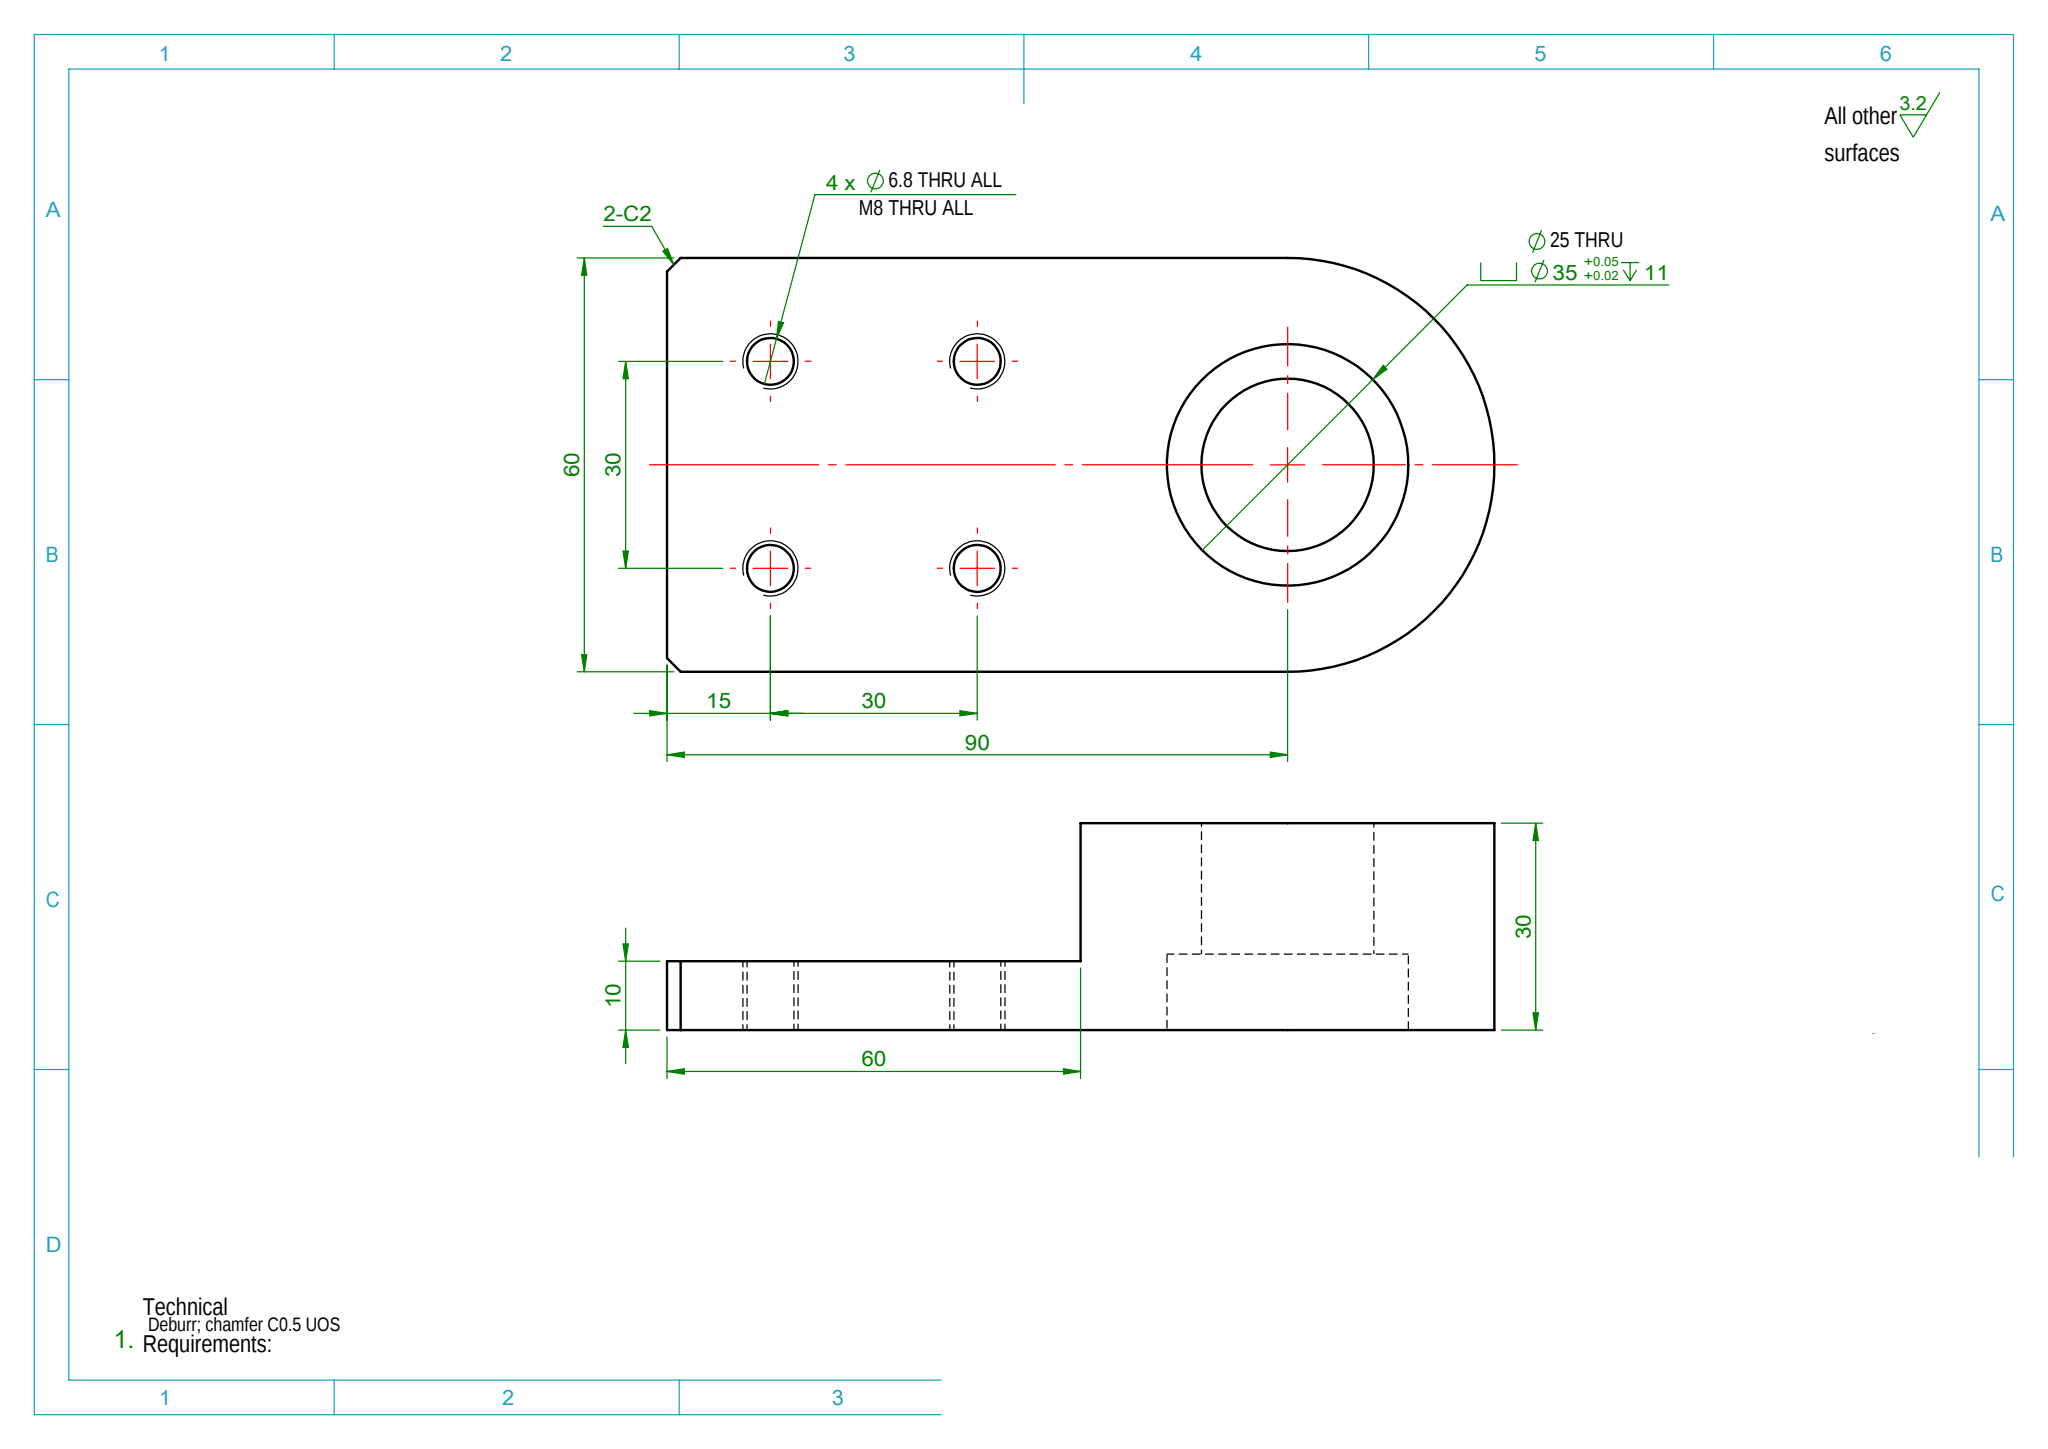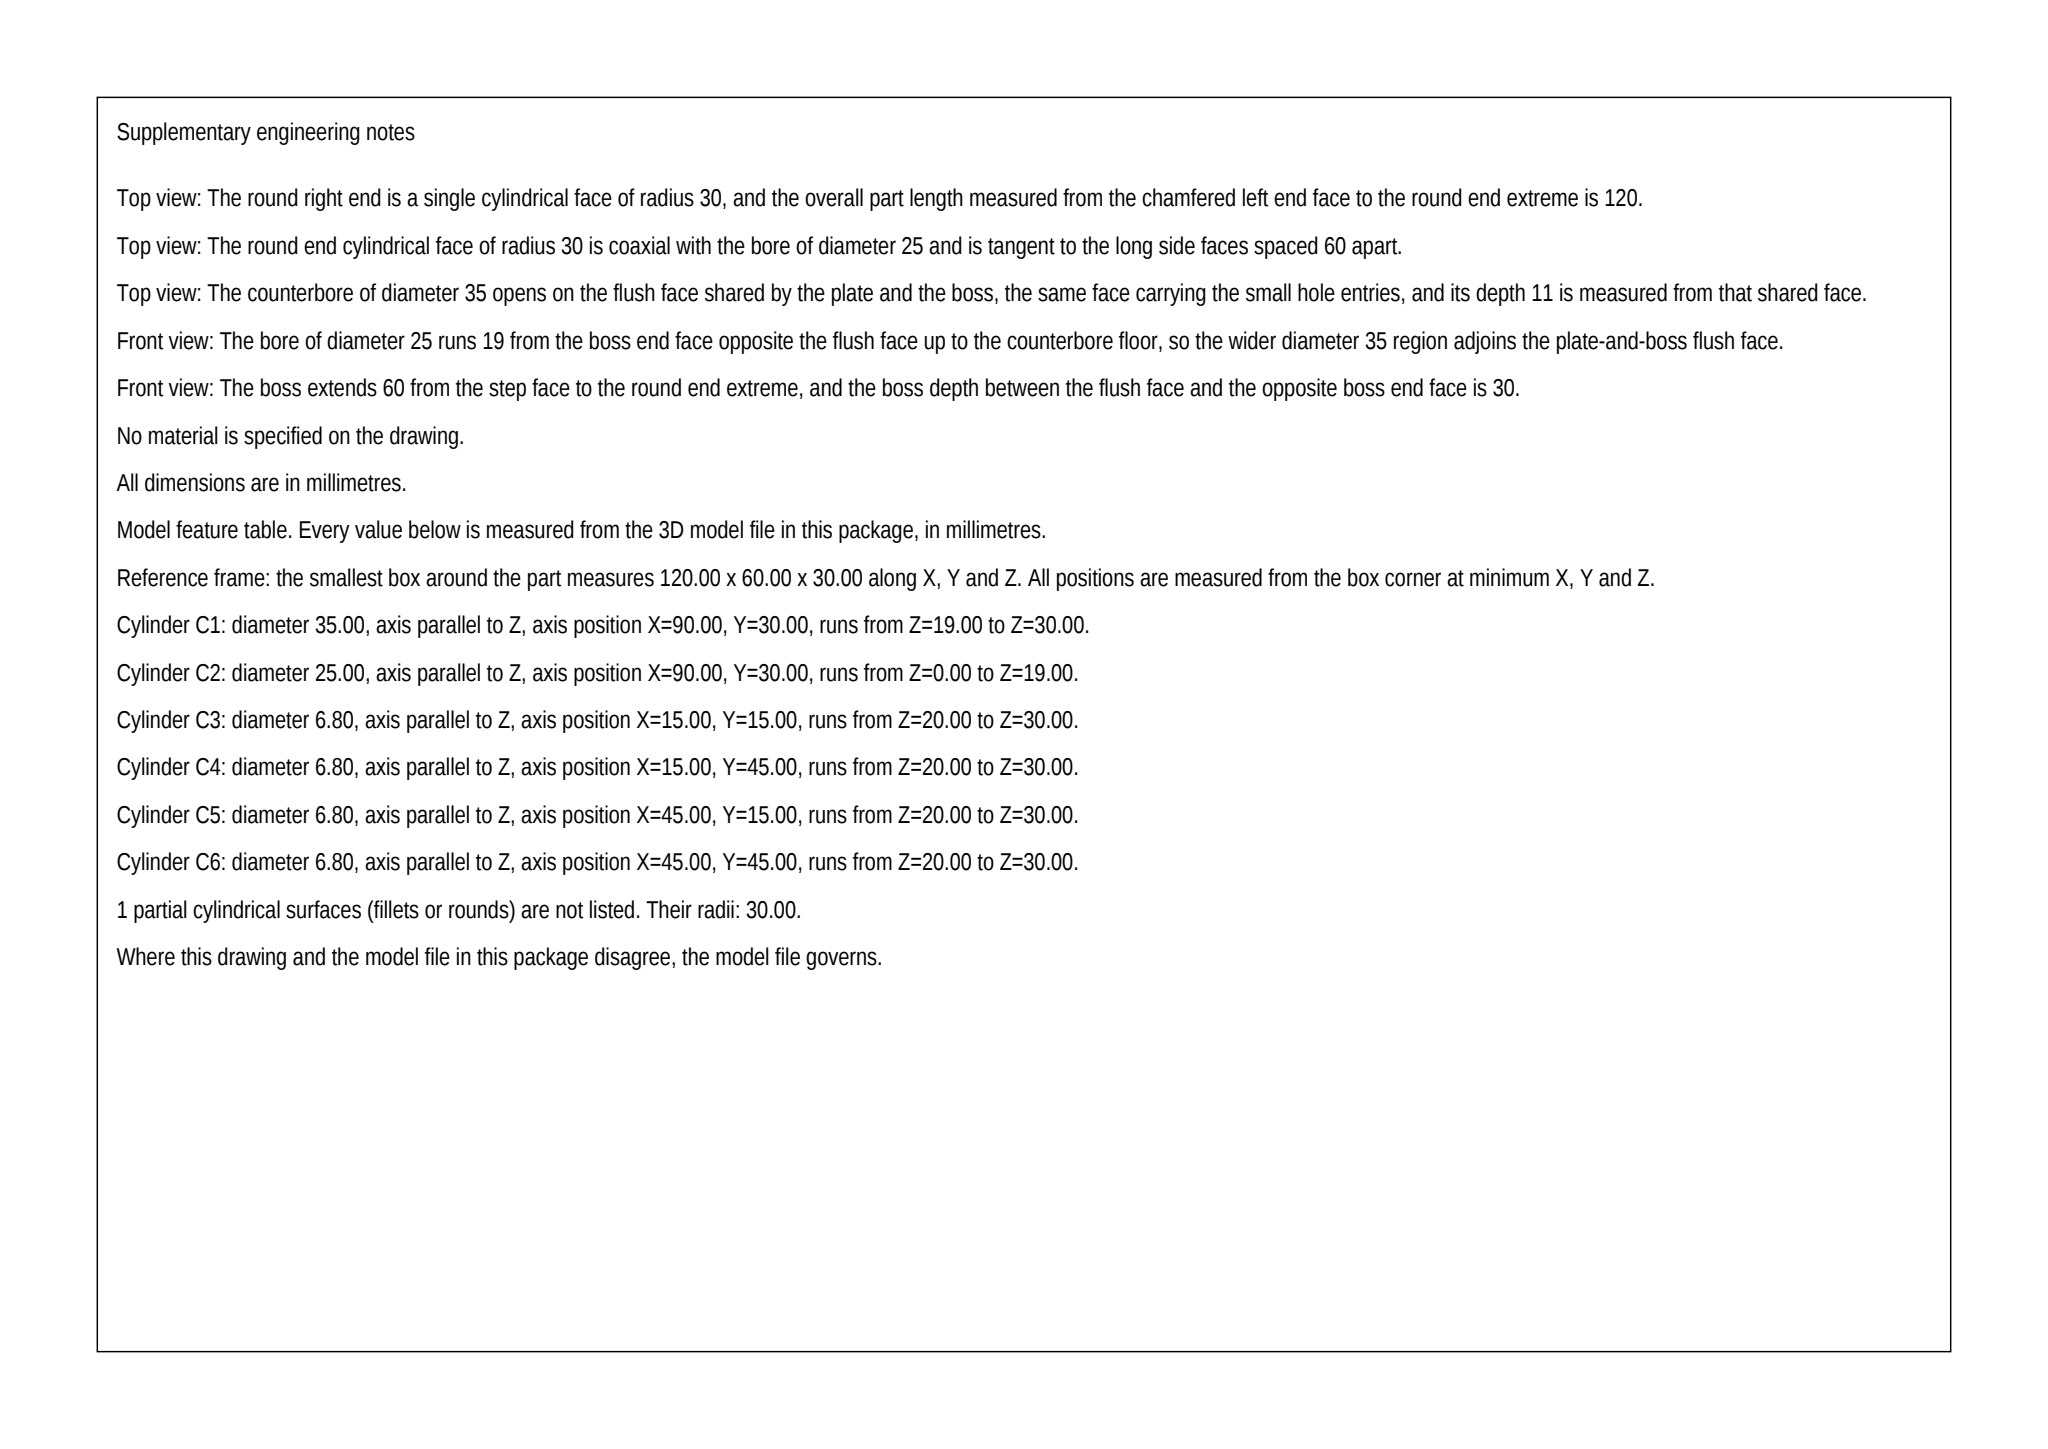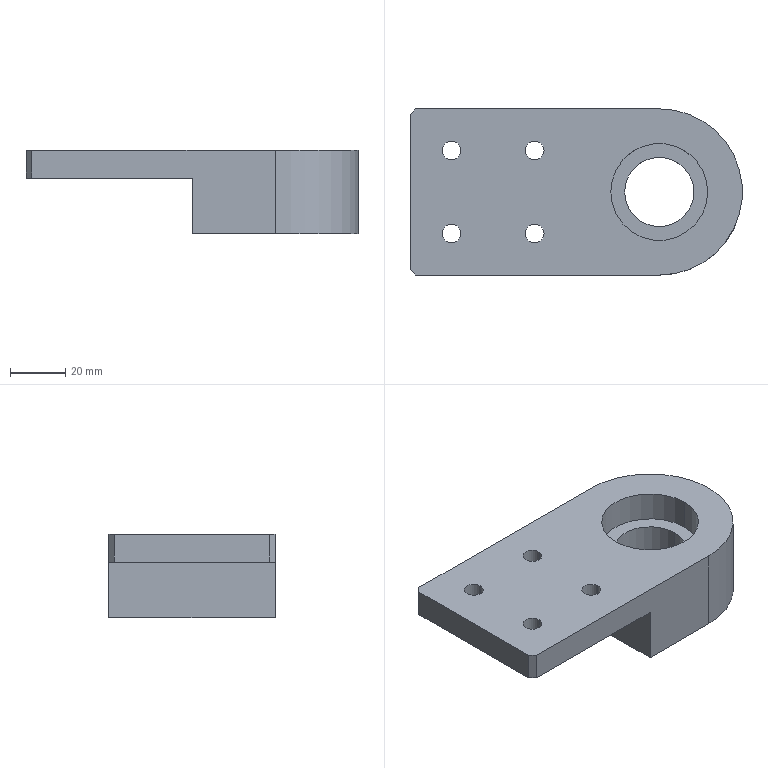Part | SolidWorks | mm | 1 solid | 23 faces | box 120 x 60 x 30 mm | volume 111009 mm3 | cylinder 13 | plane 10 | commonest cylinder face diameters 6.8 x8 25 x2 35 x2 60 x1
Drawing notes:
END ARC: R30 THRU (Ø60), C/L 90 FROM LEFT EDGE | from the solid: cylinder dia 60.0, axis z, pos (90.0,30.0), length 30.0 = full height
build123d program:
from build123d import *

# Parameters (mm, degrees)
BOSS_EXTRUDE1_DEPTH = 30
SKETCH2_W           = 60
SKETCH2_H           = 60
CUT_EXTRUDE1_DEPTH  = 20
SKETCH3_R           = 17.5
CUT_EXTRUDE2_DEPTH  = 11
SKETCH4_R           = 12.5
CUT_EXTRUDE3_DEPTH  = 83.982
M8_TAPPED_HOLE1_D   = 6.8
CHAMFER1_SIZE       = 2


with BuildPart() as part:
    # Sketch1 → Boss-Extrude1 (new body)
    with BuildSketch(Plane.XY):
        with BuildLine():
            Line((-45, 30), (45, 30))
            ThreePointArc((45, 30), (75, 0), (45, -30))
            Line((45, -30), (-45, -30))
            Line((-45, -30), (-45, 30))
        make_face()
    extrude(amount=BOSS_EXTRUDE1_DEPTH)

    # Sketch2 → Cut-Extrude1 (cut)
    with BuildSketch(Plane(origin=(0, 0, 0), x_dir=(-1, 0, 0), z_dir=(0, 0, -1))):
        with Locations((15, 0)):
            Rectangle(SKETCH2_W, SKETCH2_H)
    extrude(amount=-CUT_EXTRUDE1_DEPTH, mode=Mode.SUBTRACT)

    # Sketch3 → Cut-Extrude2 (cut)
    with BuildSketch(Plane.XY.offset(30)):
        with Locations((45, 0)):
            Circle(SKETCH3_R)
    extrude(amount=-CUT_EXTRUDE2_DEPTH, mode=Mode.SUBTRACT)

    # Sketch4 → Cut-Extrude3 (cut, through all)
    with BuildSketch(Plane.XY.offset(19)):
        with Locations((45, 0)):
            Circle(SKETCH4_R)
    extrude(amount=-CUT_EXTRUDE3_DEPTH, mode=Mode.SUBTRACT)

    # M8 Tapped Hole1 (through all)
    with Locations(Plane(origin=(0, 0, 20), x_dir=(-1, 0, 0), z_dir=(0, 0, -1))):
        with Locations((0, 15), (30, 15), (0, -15), (30, -15)):
            Hole(M8_TAPPED_HOLE1_D / 2)

    # Chamfer1
    chamfer1_edges = [part.edges().sort_by_distance(p)[0] for p in [
        (-45, -30, 25),
        (-45, 30, 25),
    ]]
    chamfer(chamfer1_edges, length=CHAMFER1_SIZE)


solid = part.part
STEP:
#1=CARTESIAN_POINT('',(3.4,15.,30.));
#2=VERTEX_POINT('',#1);
#3=CARTESIAN_POINT('',(-3.4,15.,30.));
#4=VERTEX_POINT('',#3);
#5=CARTESIAN_POINT('',(0.,15.,30.));
#6=DIRECTION('',(0.,0.,-1.));
#7=DIRECTION('',(-1.,0.,0.));
#8=AXIS2_PLACEMENT_3D('',#5,#6,#7);
#9=CIRCLE('',#8,3.4);
#10=EDGE_CURVE('',#2,#4,#9,.T.);
#11=ORIENTED_EDGE('',*,*,#10,.F.);
#12=CARTESIAN_POINT('',(3.4,15.,20.));
#13=VERTEX_POINT('',#12);
#14=CARTESIAN_POINT('',(3.4,15.,20.));
#15=DIRECTION('',(0.,0.,-1.));
#16=VECTOR('',#15,1000.);
#17=LINE('',#14,#16);
#18=EDGE_CURVE('',#2,#13,#17,.T.);
#19=ORIENTED_EDGE('',*,*,#18,.T.);
#20=CARTESIAN_POINT('',(-3.4,15.,20.));
#21=VERTEX_POINT('',#20);
#22=CARTESIAN_POINT('',(0.,15.,20.));
#23=DIRECTION('',(0.,0.,-1.));
#24=DIRECTION('',(-1.,0.,0.));
#25=AXIS2_PLACEMENT_3D('',#22,#23,#24);
#26=CIRCLE('',#25,3.4);
#27=EDGE_CURVE('',#13,#21,#26,.T.);
#28=ORIENTED_EDGE('',*,*,#27,.T.);
#29=CARTESIAN_POINT('',(-3.4,15.,20.));
#30=DIRECTION('',(0.,0.,-1.));
#31=VECTOR('',#30,1000.);
#32=LINE('',#29,#31);
#33=EDGE_CURVE('',#4,#21,#32,.T.);
#34=ORIENTED_EDGE('',*,*,#33,.F.);
#35=EDGE_LOOP('',(#11,#19,#28,#34));
#36=FACE_OUTER_BOUND('',#35,.T.);
#37=CARTESIAN_POINT('',(0.,15.,20.));
#38=DIRECTION('',(0.,0.,-1.));
#39=DIRECTION('',(-1.,0.,0.));
#40=AXIS2_PLACEMENT_3D('',#37,#38,#39);
#41=CYLINDRICAL_SURFACE('',#40,3.4);
#42=ADVANCED_FACE('',(#36),#41,.F.);
#43=CARTESIAN_POINT('',(-26.6,15.,30.));
#44=VERTEX_POINT('',#43);
#45=CARTESIAN_POINT('',(-33.4,15.,30.));
#46=VERTEX_POINT('',#45);
#47=CARTESIAN_POINT('',(-30.,15.,30.));
#48=DIRECTION('',(0.,0.,-1.));
#49=DIRECTION('',(-1.,0.,0.));
#50=AXIS2_PLACEMENT_3D('',#47,#48,#49);
#51=CIRCLE('',#50,3.4);
#52=EDGE_CURVE('',#44,#46,#51,.T.);
#53=ORIENTED_EDGE('',*,*,#52,.F.);
#54=CARTESIAN_POINT('',(-26.6,15.,20.));
#55=VERTEX_POINT('',#54);
#56=CARTESIAN_POINT('',(-26.6,15.,20.));
#57=DIRECTION('',(0.,0.,-1.));
#58=VECTOR('',#57,1000.);
#59=LINE('',#56,#58);
#60=EDGE_CURVE('',#44,#55,#59,.T.);
#61=ORIENTED_EDGE('',*,*,#60,.T.);
#62=CARTESIAN_POINT('',(-33.4,15.,20.));
#63=VERTEX_POINT('',#62);
#64=CARTESIAN_POINT('',(-30.,15.,20.));
#65=DIRECTION('',(0.,0.,-1.));
#66=DIRECTION('',(-1.,0.,0.));
#67=AXIS2_PLACEMENT_3D('',#64,#65,#66);
#68=CIRCLE('',#67,3.4);
#69=EDGE_CURVE('',#55,#63,#68,.T.);
#70=ORIENTED_EDGE('',*,*,#69,.T.);
#71=CARTESIAN_POINT('',(-33.4,15.,20.));
#72=DIRECTION('',(0.,0.,-1.));
#73=VECTOR('',#72,1000.);
#74=LINE('',#71,#73);
#75=EDGE_CURVE('',#46,#63,#74,.T.);
#76=ORIENTED_EDGE('',*,*,#75,.F.);
#77=EDGE_LOOP('',(#53,#61,#70,#76));
#78=FACE_OUTER_BOUND('',#77,.T.);
#79=CARTESIAN_POINT('',(-30.,15.,20.));
#80=DIRECTION('',(0.,0.,-1.));
#81=DIRECTION('',(-1.,0.,0.));
#82=AXIS2_PLACEMENT_3D('',#79,#80,#81);
#83=CYLINDRICAL_SURFACE('',#82,3.4);
#84=ADVANCED_FACE('',(#78),#83,.F.);
#85=CARTESIAN_POINT('',(3.4,-15.,30.));
#86=VERTEX_POINT('',#85);
#87=CARTESIAN_POINT('',(-3.4,-15.,30.));
#88=VERTEX_POINT('',#87);
#89=CARTESIAN_POINT('',(0.,-15.,30.));
#90=DIRECTION('',(0.,0.,-1.));
#91=DIRECTION('',(-1.,0.,0.));
#92=AXIS2_PLACEMENT_3D('',#89,#90,#91);
#93=CIRCLE('',#92,3.4);
#94=EDGE_CURVE('',#86,#88,#93,.T.);
#95=ORIENTED_EDGE('',*,*,#94,.F.);
#96=CARTESIAN_POINT('',(3.4,-15.,20.));
#97=VERTEX_POINT('',#96);
#98=CARTESIAN_POINT('',(3.4,-15.,20.));
#99=DIRECTION('',(0.,0.,-1.));
#100=VECTOR('',#99,1000.);
#101=LINE('',#98,#100);
#102=EDGE_CURVE('',#86,#97,#101,.T.);
#103=ORIENTED_EDGE('',*,*,#102,.T.);
#104=CARTESIAN_POINT('',(-3.4,-15.,20.));
#105=VERTEX_POINT('',#104);
#106=CARTESIAN_POINT('',(0.,-15.,20.));
#107=DIRECTION('',(0.,0.,-1.));
#108=DIRECTION('',(-1.,0.,0.));
#109=AXIS2_PLACEMENT_3D('',#106,#107,#108);
#110=CIRCLE('',#109,3.4);
#111=EDGE_CURVE('',#97,#105,#110,.T.);
#112=ORIENTED_EDGE('',*,*,#111,.T.);
#113=CARTESIAN_POINT('',(-3.4,-15.,20.));
#114=DIRECTION('',(0.,0.,-1.));
#115=VECTOR('',#114,1000.);
#116=LINE('',#113,#115);
#117=EDGE_CURVE('',#88,#105,#116,.T.);
#118=ORIENTED_EDGE('',*,*,#117,.F.);
#119=EDGE_LOOP('',(#95,#103,#112,#118));
#120=FACE_OUTER_BOUND('',#119,.T.);
#121=CARTESIAN_POINT('',(0.,-15.,20.));
#122=DIRECTION('',(0.,0.,-1.));
#123=DIRECTION('',(-1.,0.,0.));
#124=AXIS2_PLACEMENT_3D('',#121,#122,#123);
#125=CYLINDRICAL_SURFACE('',#124,3.4);
#126=ADVANCED_FACE('',(#120),#125,.F.);
#127=CARTESIAN_POINT('',(-26.6,-15.,30.));
#128=VERTEX_POINT('',#127);
#129=CARTESIAN_POINT('',(-33.4,-15.,30.));
#130=VERTEX_POINT('',#129);
#131=CARTESIAN_POINT('',(-30.,-15.,30.));
#132=DIRECTION('',(0.,0.,-1.));
#133=DIRECTION('',(-1.,0.,0.));
#134=AXIS2_PLACEMENT_3D('',#131,#132,#133);
#135=CIRCLE('',#134,3.4);
#136=EDGE_CURVE('',#128,#130,#135,.T.);
#137=ORIENTED_EDGE('',*,*,#136,.F.);
#138=CARTESIAN_POINT('',(-26.6,-15.,20.));
#139=VERTEX_POINT('',#138);
#140=CARTESIAN_POINT('',(-26.6,-15.,20.));
#141=DIRECTION('',(0.,0.,-1.));
#142=VECTOR('',#141,1000.);
#143=LINE('',#140,#142);
#144=EDGE_CURVE('',#128,#139,#143,.T.);
#145=ORIENTED_EDGE('',*,*,#144,.T.);
#146=CARTESIAN_POINT('',(-33.4,-15.,20.));
#147=VERTEX_POINT('',#146);
#148=CARTESIAN_POINT('',(-30.,-15.,20.));
#149=DIRECTION('',(0.,0.,-1.));
#150=DIRECTION('',(-1.,0.,0.));
#151=AXIS2_PLACEMENT_3D('',#148,#149,#150);
#152=CIRCLE('',#151,3.4);
#153=EDGE_CURVE('',#139,#147,#152,.T.);
#154=ORIENTED_EDGE('',*,*,#153,.T.);
#155=CARTESIAN_POINT('',(-33.4,-15.,20.));
#156=DIRECTION('',(0.,0.,-1.));
#157=VECTOR('',#156,1000.);
#158=LINE('',#155,#157);
#159=EDGE_CURVE('',#130,#147,#158,.T.);
#160=ORIENTED_EDGE('',*,*,#159,.F.);
#161=EDGE_LOOP('',(#137,#145,#154,#160));
#162=FACE_OUTER_BOUND('',#161,.T.);
#163=CARTESIAN_POINT('',(-30.,-15.,20.));
#164=DIRECTION('',(0.,0.,-1.));
#165=DIRECTION('',(-1.,0.,0.));
#166=AXIS2_PLACEMENT_3D('',#163,#164,#165);
#167=CYLINDRICAL_SURFACE('',#166,3.4);
#168=ADVANCED_FACE('',(#162),#167,.F.);
#169=CARTESIAN_POINT('',(32.5,0.,0.));
#170=VERTEX_POINT('',#169);
#171=CARTESIAN_POINT('',(57.5,0.,0.));
#172=VERTEX_POINT('',#171);
#173=CARTESIAN_POINT('',(45.,0.,0.));
#174=DIRECTION('',(0.,0.,1.));
#175=DIRECTION('',(1.,0.,0.));
#176=AXIS2_PLACEMENT_3D('',#173,#174,#175);
#177=CIRCLE('',#176,12.5);
#178=EDGE_CURVE('',#170,#172,#177,.T.);
#179=ORIENTED_EDGE('',*,*,#178,.F.);
#180=CARTESIAN_POINT('',(32.5,0.,19.));
#181=VERTEX_POINT('',#180);
#182=CARTESIAN_POINT('',(32.5,0.,0.));
#183=DIRECTION('',(0.,0.,1.));
#184=VECTOR('',#183,1000.);
#185=LINE('',#182,#184);
#186=EDGE_CURVE('',#170,#181,#185,.T.);
#187=ORIENTED_EDGE('',*,*,#186,.T.);
#188=CARTESIAN_POINT('',(57.5,0.,19.));
#189=VERTEX_POINT('',#188);
#190=CARTESIAN_POINT('',(45.,0.,19.));
#191=DIRECTION('',(0.,0.,1.));
#192=DIRECTION('',(1.,0.,0.));
#193=AXIS2_PLACEMENT_3D('',#190,#191,#192);
#194=CIRCLE('',#193,12.5);
#195=EDGE_CURVE('',#181,#189,#194,.T.);
#196=ORIENTED_EDGE('',*,*,#195,.T.);
#197=CARTESIAN_POINT('',(57.5,0.,0.));
#198=DIRECTION('',(0.,0.,1.));
#199=VECTOR('',#198,1000.);
#200=LINE('',#197,#199);
#201=EDGE_CURVE('',#172,#189,#200,.T.);
#202=ORIENTED_EDGE('',*,*,#201,.F.);
#203=EDGE_LOOP('',(#179,#187,#196,#202));
#204=FACE_OUTER_BOUND('',#203,.T.);
#205=CARTESIAN_POINT('',(45.,0.,0.));
#206=DIRECTION('',(0.,0.,1.));
#207=DIRECTION('',(1.,0.,0.));
#208=AXIS2_PLACEMENT_3D('',#205,#206,#207);
#209=CYLINDRICAL_SURFACE('',#208,12.5);
#210=ADVANCED_FACE('',(#204),#209,.F.);
#211=CARTESIAN_POINT('',(27.5,0.,19.));
#212=VERTEX_POINT('',#211);
#213=CARTESIAN_POINT('',(62.5,0.,19.));
#214=VERTEX_POINT('',#213);
#215=CARTESIAN_POINT('',(45.,0.,19.));
#216=DIRECTION('',(0.,0.,1.));
#217=DIRECTION('',(1.,0.,0.));
#218=AXIS2_PLACEMENT_3D('',#215,#216,#217);
#219=CIRCLE('',#218,17.5);
#220=EDGE_CURVE('',#212,#214,#219,.T.);
#221=ORIENTED_EDGE('',*,*,#220,.F.);
#222=CARTESIAN_POINT('',(27.5,0.,30.));
#223=VERTEX_POINT('',#222);
#224=CARTESIAN_POINT('',(27.5,0.,19.));
#225=DIRECTION('',(0.,0.,1.));
#226=VECTOR('',#225,1000.);
#227=LINE('',#224,#226);
#228=EDGE_CURVE('',#212,#223,#227,.T.);
#229=ORIENTED_EDGE('',*,*,#228,.T.);
#230=CARTESIAN_POINT('',(62.5,0.,30.));
#231=VERTEX_POINT('',#230);
#232=CARTESIAN_POINT('',(45.,0.,30.));
#233=DIRECTION('',(0.,0.,1.));
#234=DIRECTION('',(1.,0.,0.));
#235=AXIS2_PLACEMENT_3D('',#232,#233,#234);
#236=CIRCLE('',#235,17.5);
#237=EDGE_CURVE('',#223,#231,#236,.T.);
#238=ORIENTED_EDGE('',*,*,#237,.T.);
#239=CARTESIAN_POINT('',(62.5,0.,19.));
#240=DIRECTION('',(0.,0.,1.));
#241=VECTOR('',#240,1000.);
#242=LINE('',#239,#241);
#243=EDGE_CURVE('',#214,#231,#242,.T.);
#244=ORIENTED_EDGE('',*,*,#243,.F.);
#245=EDGE_LOOP('',(#221,#229,#238,#244));
#246=FACE_OUTER_BOUND('',#245,.T.);
#247=CARTESIAN_POINT('',(45.,0.,19.));
#248=DIRECTION('',(0.,0.,1.));
#249=DIRECTION('',(1.,0.,0.));
#250=AXIS2_PLACEMENT_3D('',#247,#248,#249);
#251=CYLINDRICAL_SURFACE('',#250,17.5);
#252=ADVANCED_FACE('',(#246),#251,.F.);
#253=CARTESIAN_POINT('',(-45.,-28.,20.));
#254=VERTEX_POINT('',#253);
#255=CARTESIAN_POINT('',(-45.,28.,20.));
#256=VERTEX_POINT('',#255);
#257=CARTESIAN_POINT('',(-45.,-30.,20.));
#258=DIRECTION('',(0.,1.,0.));
#259=VECTOR('',#258,1000.);
#260=LINE('',#257,#259);
#261=EDGE_CURVE('',#254,#256,#260,.T.);
#262=ORIENTED_EDGE('',*,*,#261,.F.);
#263=CARTESIAN_POINT('',(-45.,-28.,30.));
#264=VERTEX_POINT('',#263);
#265=CARTESIAN_POINT('',(-45.,-28.,30.));
#266=DIRECTION('',(0.,0.,1.));
#267=VECTOR('',#266,1000.);
#268=LINE('',#265,#267);
#269=EDGE_CURVE('',#254,#264,#268,.T.);
#270=ORIENTED_EDGE('',*,*,#269,.T.);
#271=CARTESIAN_POINT('',(-45.,28.,30.));
#272=VERTEX_POINT('',#271);
#273=CARTESIAN_POINT('',(-45.,30.,30.));
#274=DIRECTION('',(0.,-1.,0.));
#275=VECTOR('',#274,1000.);
#276=LINE('',#273,#275);
#277=EDGE_CURVE('',#272,#264,#276,.T.);
#278=ORIENTED_EDGE('',*,*,#277,.F.);
#279=CARTESIAN_POINT('',(-45.,28.,30.));
#280=DIRECTION('',(0.,0.,-1.));
#281=VECTOR('',#280,1000.);
#282=LINE('',#279,#281);
#283=EDGE_CURVE('',#272,#256,#282,.T.);
#284=ORIENTED_EDGE('',*,*,#283,.T.);
#285=EDGE_LOOP('',(#262,#270,#278,#284));
#286=FACE_OUTER_BOUND('',#285,.T.);
#287=CARTESIAN_POINT('',(-45.,30.,30.));
#288=DIRECTION('',(1.,0.,0.));
#289=DIRECTION('',(0.,0.,-1.));
#290=AXIS2_PLACEMENT_3D('',#287,#288,#289);
#291=PLANE('',#290);
#292=ADVANCED_FACE('',(#286),#291,.F.);
#293=CARTESIAN_POINT('',(45.,-30.,0.));
#294=VERTEX_POINT('',#293);
#295=CARTESIAN_POINT('',(45.,30.,0.));
#296=VERTEX_POINT('',#295);
#297=CARTESIAN_POINT('',(45.,0.,0.));
#298=DIRECTION('',(0.,0.,1.));
#299=DIRECTION('',(1.,0.,0.));
#300=AXIS2_PLACEMENT_3D('',#297,#298,#299);
#301=CIRCLE('',#300,30.);
#302=EDGE_CURVE('',#294,#296,#301,.T.);
#303=ORIENTED_EDGE('',*,*,#302,.T.);
#304=CARTESIAN_POINT('',(45.,30.,30.));
#305=VERTEX_POINT('',#304);
#306=CARTESIAN_POINT('',(45.,30.,30.));
#307=DIRECTION('',(0.,0.,-1.));
#308=VECTOR('',#307,1000.);
#309=LINE('',#306,#308);
#310=EDGE_CURVE('',#305,#296,#309,.T.);
#311=ORIENTED_EDGE('',*,*,#310,.F.);
#312=CARTESIAN_POINT('',(45.,-30.,30.));
#313=VERTEX_POINT('',#312);
#314=CARTESIAN_POINT('',(45.,0.,30.));
#315=DIRECTION('',(0.,0.,1.));
#316=DIRECTION('',(1.,0.,0.));
#317=AXIS2_PLACEMENT_3D('',#314,#315,#316);
#318=CIRCLE('',#317,30.);
#319=EDGE_CURVE('',#313,#305,#318,.T.);
#320=ORIENTED_EDGE('',*,*,#319,.F.);
#321=CARTESIAN_POINT('',(45.,-30.,30.));
#322=DIRECTION('',(0.,0.,-1.));
#323=VECTOR('',#322,1000.);
#324=LINE('',#321,#323);
#325=EDGE_CURVE('',#313,#294,#324,.T.);
#326=ORIENTED_EDGE('',*,*,#325,.T.);
#327=EDGE_LOOP('',(#303,#311,#320,#326));
#328=FACE_OUTER_BOUND('',#327,.T.);
#329=CARTESIAN_POINT('',(45.,0.,30.));
#330=DIRECTION('',(0.,0.,-1.));
#331=DIRECTION('',(-1.,0.,0.));
#332=AXIS2_PLACEMENT_3D('',#329,#330,#331);
#333=CYLINDRICAL_SURFACE('',#332,30.);
#334=ADVANCED_FACE('',(#328),#333,.T.);
#335=CARTESIAN_POINT('',(-43.,30.,20.));
#336=VERTEX_POINT('',#335);
#337=CARTESIAN_POINT('',(15.,30.,20.));
#338=VERTEX_POINT('',#337);
#339=CARTESIAN_POINT('',(-45.,30.,20.));
#340=DIRECTION('',(1.,0.,0.));
#341=VECTOR('',#340,1000.);
#342=LINE('',#339,#341);
#343=EDGE_CURVE('',#336,#338,#342,.T.);
#344=ORIENTED_EDGE('',*,*,#343,.F.);
#345=CARTESIAN_POINT('',(-43.,30.,30.));
#346=VERTEX_POINT('',#345);
#347=CARTESIAN_POINT('',(-43.,30.,30.));
#348=DIRECTION('',(0.,0.,1.));
#349=VECTOR('',#348,1000.);
#350=LINE('',#347,#349);
#351=EDGE_CURVE('',#336,#346,#350,.T.);
#352=ORIENTED_EDGE('',*,*,#351,.T.);
#353=CARTESIAN_POINT('',(-45.,30.,30.));
#354=DIRECTION('',(-1.,0.,0.));
#355=VECTOR('',#354,1000.);
#356=LINE('',#353,#355);
#357=EDGE_CURVE('',#305,#346,#356,.T.);
#358=ORIENTED_EDGE('',*,*,#357,.F.);
#359=ORIENTED_EDGE('',*,*,#310,.T.);
#360=CARTESIAN_POINT('',(15.,30.,0.));
#361=VERTEX_POINT('',#360);
#362=CARTESIAN_POINT('',(-45.,30.,0.));
#363=DIRECTION('',(-1.,0.,0.));
#364=VECTOR('',#363,1000.);
#365=LINE('',#362,#364);
#366=EDGE_CURVE('',#296,#361,#365,.T.);
#367=ORIENTED_EDGE('',*,*,#366,.T.);
#368=CARTESIAN_POINT('',(15.,30.,20.));
#369=DIRECTION('',(0.,0.,-1.));
#370=VECTOR('',#369,1000.);
#371=LINE('',#368,#370);
#372=EDGE_CURVE('',#338,#361,#371,.T.);
#373=ORIENTED_EDGE('',*,*,#372,.F.);
#374=EDGE_LOOP('',(#344,#352,#358,#359,#367,#373));
#375=FACE_OUTER_BOUND('',#374,.T.);
#376=CARTESIAN_POINT('',(-45.,30.,30.));
#377=DIRECTION('',(0.,-1.,0.));
#378=DIRECTION('',(0.,0.,-1.));
#379=AXIS2_PLACEMENT_3D('',#376,#377,#378);
#380=PLANE('',#379);
#381=ADVANCED_FACE('',(#375),#380,.F.);
#382=CARTESIAN_POINT('',(-43.,-30.,30.));
#383=VERTEX_POINT('',#382);
#384=CARTESIAN_POINT('',(-45.,-30.,30.));
#385=DIRECTION('',(1.,0.,0.));
#386=VECTOR('',#385,1000.);
#387=LINE('',#384,#386);
#388=EDGE_CURVE('',#383,#313,#387,.T.);
#389=ORIENTED_EDGE('',*,*,#388,.F.);
#390=CARTESIAN_POINT('',(-43.,-30.,20.));
#391=VERTEX_POINT('',#390);
#392=CARTESIAN_POINT('',(-43.,-30.,30.));
#393=DIRECTION('',(0.,0.,-1.));
#394=VECTOR('',#393,1000.);
#395=LINE('',#392,#394);
#396=EDGE_CURVE('',#383,#391,#395,.T.);
#397=ORIENTED_EDGE('',*,*,#396,.T.);
#398=CARTESIAN_POINT('',(15.,-30.,20.));
#399=VERTEX_POINT('',#398);
#400=CARTESIAN_POINT('',(-45.,-30.,20.));
#401=DIRECTION('',(-1.,0.,0.));
#402=VECTOR('',#401,1000.);
#403=LINE('',#400,#402);
#404=EDGE_CURVE('',#399,#391,#403,.T.);
#405=ORIENTED_EDGE('',*,*,#404,.F.);
#406=CARTESIAN_POINT('',(15.,-30.,0.));
#407=VERTEX_POINT('',#406);
#408=CARTESIAN_POINT('',(15.,-30.,20.));
#409=DIRECTION('',(0.,0.,-1.));
#410=VECTOR('',#409,1000.);
#411=LINE('',#408,#410);
#412=EDGE_CURVE('',#399,#407,#411,.T.);
#413=ORIENTED_EDGE('',*,*,#412,.T.);
#414=CARTESIAN_POINT('',(-45.,-30.,0.));
#415=DIRECTION('',(1.,0.,0.));
#416=VECTOR('',#415,1000.);
#417=LINE('',#414,#416);
#418=EDGE_CURVE('',#407,#294,#417,.T.);
#419=ORIENTED_EDGE('',*,*,#418,.T.);
#420=ORIENTED_EDGE('',*,*,#325,.F.);
#421=EDGE_LOOP('',(#389,#397,#405,#413,#419,#420));
#422=FACE_OUTER_BOUND('',#421,.T.);
#423=CARTESIAN_POINT('',(-45.,-30.,30.));
#424=DIRECTION('',(0.,1.,0.));
#425=DIRECTION('',(0.,0.,1.));
#426=AXIS2_PLACEMENT_3D('',#423,#424,#425);
#427=PLANE('',#426);
#428=ADVANCED_FACE('',(#422),#427,.F.);
#429=CARTESIAN_POINT('',(0.,15.,30.));
#430=DIRECTION('',(0.,0.,-1.));
#431=DIRECTION('',(-1.,0.,0.));
#432=AXIS2_PLACEMENT_3D('',#429,#430,#431);
#433=CIRCLE('',#432,3.4);
#434=EDGE_CURVE('',#4,#2,#433,.T.);
#435=ORIENTED_EDGE('',*,*,#434,.T.);
#436=ORIENTED_EDGE('',*,*,#10,.T.);
#437=EDGE_LOOP('',(#435,#436));
#438=FACE_BOUND('',#437,.T.);
#439=CARTESIAN_POINT('',(-30.,15.,30.));
#440=DIRECTION('',(0.,0.,-1.));
#441=DIRECTION('',(-1.,0.,0.));
#442=AXIS2_PLACEMENT_3D('',#439,#440,#441);
#443=CIRCLE('',#442,3.4);
#444=EDGE_CURVE('',#46,#44,#443,.T.);
#445=ORIENTED_EDGE('',*,*,#444,.T.);
#446=ORIENTED_EDGE('',*,*,#52,.T.);
#447=EDGE_LOOP('',(#445,#446));
#448=FACE_BOUND('',#447,.T.);
#449=CARTESIAN_POINT('',(0.,-15.,30.));
#450=DIRECTION('',(0.,0.,-1.));
#451=DIRECTION('',(-1.,0.,0.));
#452=AXIS2_PLACEMENT_3D('',#449,#450,#451);
#453=CIRCLE('',#452,3.4);
#454=EDGE_CURVE('',#88,#86,#453,.T.);
#455=ORIENTED_EDGE('',*,*,#454,.T.);
#456=ORIENTED_EDGE('',*,*,#94,.T.);
#457=EDGE_LOOP('',(#455,#456));
#458=FACE_BOUND('',#457,.T.);
#459=CARTESIAN_POINT('',(-30.,-15.,30.));
#460=DIRECTION('',(0.,0.,-1.));
#461=DIRECTION('',(-1.,0.,0.));
#462=AXIS2_PLACEMENT_3D('',#459,#460,#461);
#463=CIRCLE('',#462,3.4);
#464=EDGE_CURVE('',#130,#128,#463,.T.);
#465=ORIENTED_EDGE('',*,*,#464,.T.);
#466=ORIENTED_EDGE('',*,*,#136,.T.);
#467=EDGE_LOOP('',(#465,#466));
#468=FACE_BOUND('',#467,.T.);
#469=CARTESIAN_POINT('',(45.,0.,30.));
#470=DIRECTION('',(0.,0.,1.));
#471=DIRECTION('',(1.,0.,0.));
#472=AXIS2_PLACEMENT_3D('',#469,#470,#471);
#473=CIRCLE('',#472,17.5);
#474=EDGE_CURVE('',#231,#223,#473,.T.);
#475=ORIENTED_EDGE('',*,*,#474,.F.);
#476=ORIENTED_EDGE('',*,*,#237,.F.);
#477=EDGE_LOOP('',(#475,#476));
#478=FACE_BOUND('',#477,.T.);
#479=ORIENTED_EDGE('',*,*,#277,.T.);
#480=CARTESIAN_POINT('',(-14.,-59.,30.));
#481=DIRECTION('',(0.7071,-0.7071,0.));
#482=VECTOR('',#481,1000.);
#483=LINE('',#480,#482);
#484=EDGE_CURVE('',#264,#383,#483,.T.);
#485=ORIENTED_EDGE('',*,*,#484,.T.);
#486=ORIENTED_EDGE('',*,*,#388,.T.);
#487=ORIENTED_EDGE('',*,*,#319,.T.);
#488=ORIENTED_EDGE('',*,*,#357,.T.);
#489=CARTESIAN_POINT('',(-14.,59.,30.));
#490=DIRECTION('',(-0.7071,-0.7071,0.));
#491=VECTOR('',#490,1000.);
#492=LINE('',#489,#491);
#493=EDGE_CURVE('',#346,#272,#492,.T.);
#494=ORIENTED_EDGE('',*,*,#493,.T.);
#495=EDGE_LOOP('',(#479,#485,#486,#487,#488,#494));
#496=FACE_OUTER_BOUND('',#495,.T.);
#497=CARTESIAN_POINT('',(45.,0.,30.));
#498=DIRECTION('',(0.,0.,1.));
#499=DIRECTION('',(1.,0.,0.));
#500=AXIS2_PLACEMENT_3D('',#497,#498,#499);
#501=PLANE('',#500);
#502=ADVANCED_FACE('',(#438,#448,#458,#468,#478,#496),#501,.T.);
#503=CARTESIAN_POINT('',(45.,0.,0.));
#504=DIRECTION('',(0.,0.,1.));
#505=DIRECTION('',(1.,0.,0.));
#506=AXIS2_PLACEMENT_3D('',#503,#504,#505);
#507=CIRCLE('',#506,12.5);
#508=EDGE_CURVE('',#172,#170,#507,.T.);
#509=ORIENTED_EDGE('',*,*,#508,.T.);
#510=ORIENTED_EDGE('',*,*,#178,.T.);
#511=EDGE_LOOP('',(#509,#510));
#512=FACE_BOUND('',#511,.T.);
#513=ORIENTED_EDGE('',*,*,#418,.F.);
#514=CARTESIAN_POINT('',(15.,-30.,0.));
#515=DIRECTION('',(-0.,-1.,0.));
#516=VECTOR('',#515,1000.);
#517=LINE('',#514,#516);
#518=EDGE_CURVE('',#361,#407,#517,.T.);
#519=ORIENTED_EDGE('',*,*,#518,.F.);
#520=ORIENTED_EDGE('',*,*,#366,.F.);
#521=ORIENTED_EDGE('',*,*,#302,.F.);
#522=EDGE_LOOP('',(#513,#519,#520,#521));
#523=FACE_OUTER_BOUND('',#522,.T.);
#524=CARTESIAN_POINT('',(45.,0.,0.));
#525=DIRECTION('',(0.,0.,1.));
#526=DIRECTION('',(1.,0.,0.));
#527=AXIS2_PLACEMENT_3D('',#524,#525,#526);
#528=PLANE('',#527);
#529=ADVANCED_FACE('',(#512,#523),#528,.F.);
#530=ORIENTED_EDGE('',*,*,#518,.T.);
#531=ORIENTED_EDGE('',*,*,#412,.F.);
#532=CARTESIAN_POINT('',(15.,-30.,20.));
#533=DIRECTION('',(-0.,-1.,0.));
#534=VECTOR('',#533,1000.);
#535=LINE('',#532,#534);
#536=EDGE_CURVE('',#338,#399,#535,.T.);
#537=ORIENTED_EDGE('',*,*,#536,.F.);
#538=ORIENTED_EDGE('',*,*,#372,.T.);
#539=EDGE_LOOP('',(#530,#531,#537,#538));
#540=FACE_OUTER_BOUND('',#539,.T.);
#541=CARTESIAN_POINT('',(15.,-30.,20.));
#542=DIRECTION('',(1.,-0.,0.));
#543=DIRECTION('',(0.,1.,0.));
#544=AXIS2_PLACEMENT_3D('',#541,#542,#543);
#545=PLANE('',#544);
#546=ADVANCED_FACE('',(#540),#545,.F.);
#547=CARTESIAN_POINT('',(0.,15.,20.));
#548=DIRECTION('',(0.,0.,-1.));
#549=DIRECTION('',(-1.,0.,0.));
#550=AXIS2_PLACEMENT_3D('',#547,#548,#549);
#551=CIRCLE('',#550,3.4);
#552=EDGE_CURVE('',#21,#13,#551,.T.);
#553=ORIENTED_EDGE('',*,*,#552,.F.);
#554=ORIENTED_EDGE('',*,*,#27,.F.);
#555=EDGE_LOOP('',(#553,#554));
#556=FACE_BOUND('',#555,.T.);
#557=CARTESIAN_POINT('',(-30.,15.,20.));
#558=DIRECTION('',(0.,0.,-1.));
#559=DIRECTION('',(-1.,0.,0.));
#560=AXIS2_PLACEMENT_3D('',#557,#558,#559);
#561=CIRCLE('',#560,3.4);
#562=EDGE_CURVE('',#63,#55,#561,.T.);
#563=ORIENTED_EDGE('',*,*,#562,.F.);
#564=ORIENTED_EDGE('',*,*,#69,.F.);
#565=EDGE_LOOP('',(#563,#564));
#566=FACE_BOUND('',#565,.T.);
#567=CARTESIAN_POINT('',(0.,-15.,20.));
#568=DIRECTION('',(0.,0.,-1.));
#569=DIRECTION('',(-1.,0.,0.));
#570=AXIS2_PLACEMENT_3D('',#567,#568,#569);
#571=CIRCLE('',#570,3.4);
#572=EDGE_CURVE('',#105,#97,#571,.T.);
#573=ORIENTED_EDGE('',*,*,#572,.F.);
#574=ORIENTED_EDGE('',*,*,#111,.F.);
#575=EDGE_LOOP('',(#573,#574));
#576=FACE_BOUND('',#575,.T.);
#577=CARTESIAN_POINT('',(-30.,-15.,20.));
#578=DIRECTION('',(0.,0.,-1.));
#579=DIRECTION('',(-1.,0.,0.));
#580=AXIS2_PLACEMENT_3D('',#577,#578,#579);
#581=CIRCLE('',#580,3.4);
#582=EDGE_CURVE('',#147,#139,#581,.T.);
#583=ORIENTED_EDGE('',*,*,#582,.F.);
#584=ORIENTED_EDGE('',*,*,#153,.F.);
#585=EDGE_LOOP('',(#583,#584));
#586=FACE_BOUND('',#585,.T.);
#587=ORIENTED_EDGE('',*,*,#404,.T.);
#588=CARTESIAN_POINT('',(-36.5,-36.5,20.));
#589=DIRECTION('',(-0.7071,0.7071,0.));
#590=VECTOR('',#589,1000.);
#591=LINE('',#588,#590);
#592=EDGE_CURVE('',#391,#254,#591,.T.);
#593=ORIENTED_EDGE('',*,*,#592,.T.);
#594=ORIENTED_EDGE('',*,*,#261,.T.);
#595=CARTESIAN_POINT('',(-36.5,36.5,20.));
#596=DIRECTION('',(0.7071,0.7071,0.));
#597=VECTOR('',#596,1000.);
#598=LINE('',#595,#597);
#599=EDGE_CURVE('',#256,#336,#598,.T.);
#600=ORIENTED_EDGE('',*,*,#599,.T.);
#601=ORIENTED_EDGE('',*,*,#343,.T.);
#602=ORIENTED_EDGE('',*,*,#536,.T.);
#603=EDGE_LOOP('',(#587,#593,#594,#600,#601,#602));
#604=FACE_OUTER_BOUND('',#603,.T.);
#605=CARTESIAN_POINT('',(0.,0.,20.));
#606=DIRECTION('',(0.,0.,-1.));
#607=DIRECTION('',(-1.,0.,0.));
#608=AXIS2_PLACEMENT_3D('',#605,#606,#607);
#609=PLANE('',#608);
#610=ADVANCED_FACE('',(#556,#566,#576,#586,#604),#609,.T.);
#611=ORIENTED_EDGE('',*,*,#228,.F.);
#612=CARTESIAN_POINT('',(45.,0.,19.));
#613=DIRECTION('',(0.,0.,1.));
#614=DIRECTION('',(1.,0.,0.));
#615=AXIS2_PLACEMENT_3D('',#612,#613,#614);
#616=CIRCLE('',#615,17.5);
#617=EDGE_CURVE('',#214,#212,#616,.T.);
#618=ORIENTED_EDGE('',*,*,#617,.F.);
#619=ORIENTED_EDGE('',*,*,#243,.T.);
#620=ORIENTED_EDGE('',*,*,#474,.T.);
#621=EDGE_LOOP('',(#611,#618,#619,#620));
#622=FACE_OUTER_BOUND('',#621,.T.);
#623=CARTESIAN_POINT('',(45.,0.,19.));
#624=DIRECTION('',(0.,0.,1.));
#625=DIRECTION('',(1.,0.,0.));
#626=AXIS2_PLACEMENT_3D('',#623,#624,#625);
#627=CYLINDRICAL_SURFACE('',#626,17.5);
#628=ADVANCED_FACE('',(#622),#627,.F.);
#629=CARTESIAN_POINT('',(45.,0.,19.));
#630=DIRECTION('',(0.,0.,1.));
#631=DIRECTION('',(1.,0.,0.));
#632=AXIS2_PLACEMENT_3D('',#629,#630,#631);
#633=CIRCLE('',#632,12.5);
#634=EDGE_CURVE('',#189,#181,#633,.T.);
#635=ORIENTED_EDGE('',*,*,#634,.F.);
#636=ORIENTED_EDGE('',*,*,#195,.F.);
#637=EDGE_LOOP('',(#635,#636));
#638=FACE_BOUND('',#637,.T.);
#639=ORIENTED_EDGE('',*,*,#617,.T.);
#640=ORIENTED_EDGE('',*,*,#220,.T.);
#641=EDGE_LOOP('',(#639,#640));
#642=FACE_OUTER_BOUND('',#641,.T.);
#643=CARTESIAN_POINT('',(45.,0.,19.));
#644=DIRECTION('',(0.,0.,1.));
#645=DIRECTION('',(1.,0.,0.));
#646=AXIS2_PLACEMENT_3D('',#643,#644,#645);
#647=PLANE('',#646);
#648=ADVANCED_FACE('',(#638,#642),#647,.T.);
#649=ORIENTED_EDGE('',*,*,#186,.F.);
#650=ORIENTED_EDGE('',*,*,#508,.F.);
#651=ORIENTED_EDGE('',*,*,#201,.T.);
#652=ORIENTED_EDGE('',*,*,#634,.T.);
#653=EDGE_LOOP('',(#649,#650,#651,#652));
#654=FACE_OUTER_BOUND('',#653,.T.);
#655=CARTESIAN_POINT('',(45.,0.,0.));
#656=DIRECTION('',(0.,0.,1.));
#657=DIRECTION('',(1.,0.,0.));
#658=AXIS2_PLACEMENT_3D('',#655,#656,#657);
#659=CYLINDRICAL_SURFACE('',#658,12.5);
#660=ADVANCED_FACE('',(#654),#659,.F.);
#661=ORIENTED_EDGE('',*,*,#144,.F.);
#662=ORIENTED_EDGE('',*,*,#464,.F.);
#663=ORIENTED_EDGE('',*,*,#159,.T.);
#664=ORIENTED_EDGE('',*,*,#582,.T.);
#665=EDGE_LOOP('',(#661,#662,#663,#664));
#666=FACE_OUTER_BOUND('',#665,.T.);
#667=CARTESIAN_POINT('',(-30.,-15.,20.));
#668=DIRECTION('',(0.,0.,-1.));
#669=DIRECTION('',(-1.,0.,0.));
#670=AXIS2_PLACEMENT_3D('',#667,#668,#669);
#671=CYLINDRICAL_SURFACE('',#670,3.4);
#672=ADVANCED_FACE('',(#666),#671,.F.);
#673=ORIENTED_EDGE('',*,*,#102,.F.);
#674=ORIENTED_EDGE('',*,*,#454,.F.);
#675=ORIENTED_EDGE('',*,*,#117,.T.);
#676=ORIENTED_EDGE('',*,*,#572,.T.);
#677=EDGE_LOOP('',(#673,#674,#675,#676));
#678=FACE_OUTER_BOUND('',#677,.T.);
#679=CARTESIAN_POINT('',(0.,-15.,20.));
#680=DIRECTION('',(0.,0.,-1.));
#681=DIRECTION('',(-1.,0.,0.));
#682=AXIS2_PLACEMENT_3D('',#679,#680,#681);
#683=CYLINDRICAL_SURFACE('',#682,3.4);
#684=ADVANCED_FACE('',(#678),#683,.F.);
#685=ORIENTED_EDGE('',*,*,#60,.F.);
#686=ORIENTED_EDGE('',*,*,#444,.F.);
#687=ORIENTED_EDGE('',*,*,#75,.T.);
#688=ORIENTED_EDGE('',*,*,#562,.T.);
#689=EDGE_LOOP('',(#685,#686,#687,#688));
#690=FACE_OUTER_BOUND('',#689,.T.);
#691=CARTESIAN_POINT('',(-30.,15.,20.));
#692=DIRECTION('',(0.,0.,-1.));
#693=DIRECTION('',(-1.,0.,0.));
#694=AXIS2_PLACEMENT_3D('',#691,#692,#693);
#695=CYLINDRICAL_SURFACE('',#694,3.4);
#696=ADVANCED_FACE('',(#690),#695,.F.);
#697=ORIENTED_EDGE('',*,*,#18,.F.);
#698=ORIENTED_EDGE('',*,*,#434,.F.);
#699=ORIENTED_EDGE('',*,*,#33,.T.);
#700=ORIENTED_EDGE('',*,*,#552,.T.);
#701=EDGE_LOOP('',(#697,#698,#699,#700));
#702=FACE_OUTER_BOUND('',#701,.T.);
#703=CARTESIAN_POINT('',(0.,15.,20.));
#704=DIRECTION('',(0.,0.,-1.));
#705=DIRECTION('',(-1.,0.,0.));
#706=AXIS2_PLACEMENT_3D('',#703,#704,#705);
#707=CYLINDRICAL_SURFACE('',#706,3.4);
#708=ADVANCED_FACE('',(#702),#707,.F.);
#709=ORIENTED_EDGE('',*,*,#484,.F.);
#710=ORIENTED_EDGE('',*,*,#269,.F.);
#711=ORIENTED_EDGE('',*,*,#592,.F.);
#712=ORIENTED_EDGE('',*,*,#396,.F.);
#713=EDGE_LOOP('',(#709,#710,#711,#712));
#714=FACE_OUTER_BOUND('',#713,.T.);
#715=CARTESIAN_POINT('',(-43.,-30.,30.));
#716=DIRECTION('',(0.7071,0.7071,0.));
#717=DIRECTION('',(0.,0.,-1.));
#718=AXIS2_PLACEMENT_3D('',#715,#716,#717);
#719=PLANE('',#718);
#720=ADVANCED_FACE('',(#714),#719,.F.);
#721=ORIENTED_EDGE('',*,*,#493,.F.);
#722=ORIENTED_EDGE('',*,*,#351,.F.);
#723=ORIENTED_EDGE('',*,*,#599,.F.);
#724=ORIENTED_EDGE('',*,*,#283,.F.);
#725=EDGE_LOOP('',(#721,#722,#723,#724));
#726=FACE_OUTER_BOUND('',#725,.T.);
#727=CARTESIAN_POINT('',(-45.,28.,30.));
#728=DIRECTION('',(0.7071,-0.7071,0.));
#729=DIRECTION('',(0.,0.,-1.));
#730=AXIS2_PLACEMENT_3D('',#727,#728,#729);
#731=PLANE('',#730);
#732=ADVANCED_FACE('',(#726),#731,.F.);
#733=CLOSED_SHELL('',(#42,#84,#126,#168,#210,#252,#292,#334,#381,#428,#502,#529,#546,#610,#628,#648,#660,#672,#684,#696,#708,#720,#732));
#734=MANIFOLD_SOLID_BREP('',#733);
#735=CARTESIAN_POINT('',(0.,0.,0.));
#736=DIRECTION('',(0.,0.,1.));
#737=DIRECTION('',(1.,0.,0.));
#738=AXIS2_PLACEMENT_3D('',#735,#736,#737);
#739=(LENGTH_UNIT()NAMED_UNIT(*)SI_UNIT(.MILLI.,.METRE.));
#740=UNCERTAINTY_MEASURE_WITH_UNIT(LENGTH_MEASURE(0.00001),#739,'','');
#741=(NAMED_UNIT(*)PLANE_ANGLE_UNIT()SI_UNIT($,.RADIAN.));
#742=(NAMED_UNIT(*)SI_UNIT($,.STERADIAN.)SOLID_ANGLE_UNIT());
#743=(GEOMETRIC_REPRESENTATION_CONTEXT(3)GLOBAL_UNCERTAINTY_ASSIGNED_CONTEXT((#740))GLOBAL_UNIT_ASSIGNED_CONTEXT((#739,#741,#742))REPRESENTATION_CONTEXT('',''));
#744=ADVANCED_BREP_SHAPE_REPRESENTATION('',(#734,#738),#743);